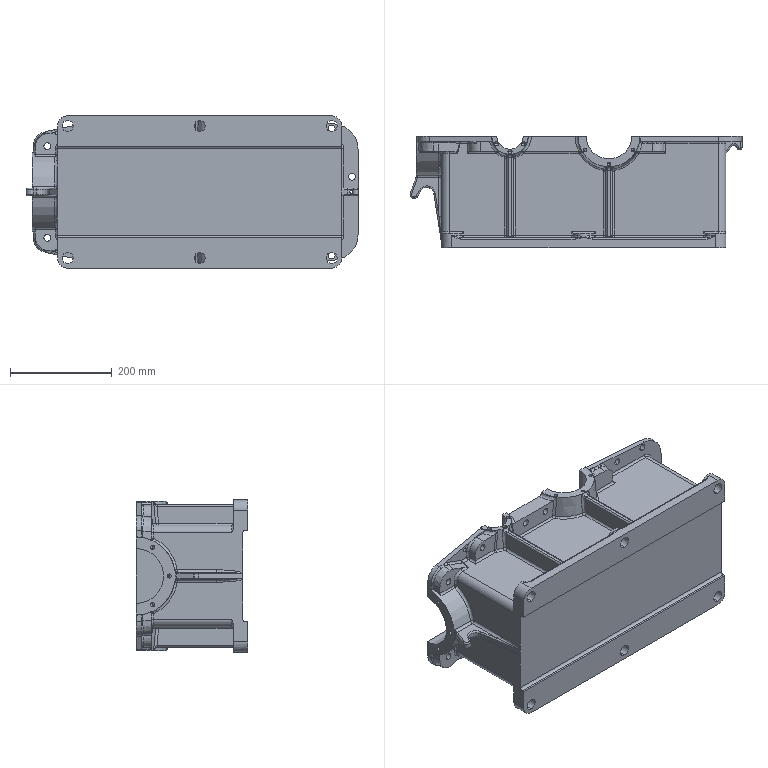Component | SolidWorks | MachineBase-1 | 1 solid | 568 faces | volume 7136061 mm3 | cylinder 226 | plane 113 | spline 97 | torus 76 | cone 44 | sphere 12 | commonest cylinder face diameters 8 x91 13.5 x26 6 x26 10 x25 22 x12 6.8 x12 40 x9 44 x4